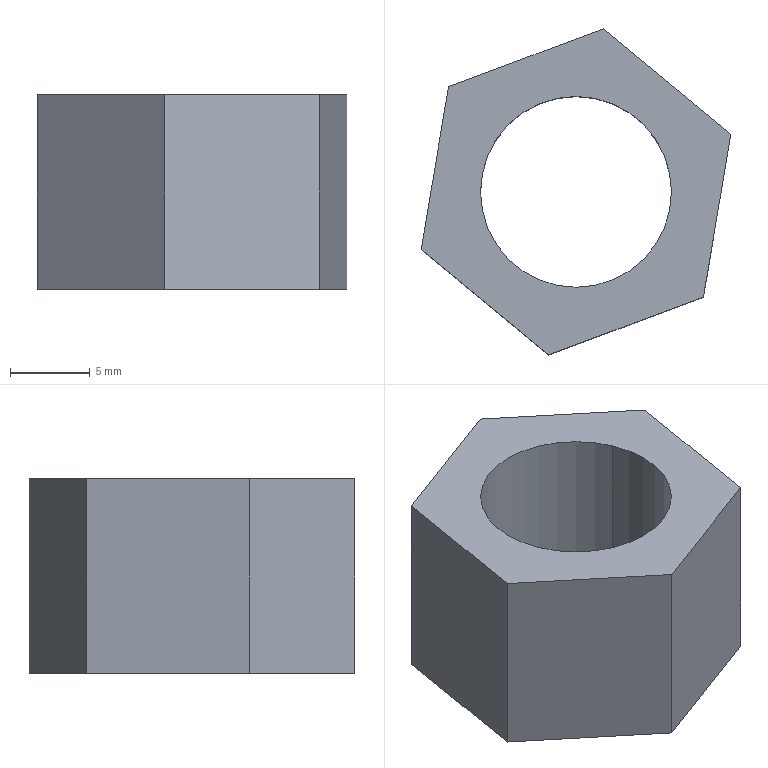Component | SolidWorks | M12Nut-2 | 1 solid | 10 faces | box 19.47 x 20.5 x 12.2 mm | volume 2043 mm3 | plane 8 | cylinder 2 | commonest cylinder face diameters 12 x2
STEP:
#1=COLOUR_RGB('',0.7922,0.8196,0.9333);
#2=FILL_AREA_STYLE_COLOUR('',#1);
#3=FILL_AREA_STYLE('',(#2));
#4=SURFACE_STYLE_FILL_AREA(#3);
#5=SURFACE_SIDE_STYLE('',(#4));
#6=SURFACE_STYLE_USAGE(.BOTH.,#5);
#7=PRESENTATION_STYLE_ASSIGNMENT((#6));
#8=CARTESIAN_POINT('',(21.066,-0.0173,0.542));
#9=VERTEX_POINT('',#8);
#10=CARTESIAN_POINT('',(20.629,-0.1983,0.542));
#11=VERTEX_POINT('',#10);
#12=CARTESIAN_POINT('',(20.847,-0.1078,0.542));
#13=DIRECTION('',(-0.,-0.,-1.));
#14=DIRECTION('',(-0.9237,-0.383,0.));
#15=AXIS2_PLACEMENT_3D('',#12,#13,#14);
#16=CIRCLE('',#15,0.2362);
#17=EDGE_CURVE('',#9,#11,#16,.T.);
#18=ORIENTED_EDGE('',*,*,#17,.F.);
#19=CARTESIAN_POINT('',(21.066,-0.0173,0.06171));
#20=VERTEX_POINT('',#19);
#21=CARTESIAN_POINT('',(21.066,-0.0173,0.5639));
#22=DIRECTION('',(-0.,-0.,-1.));
#23=VECTOR('',#22,39.37);
#24=LINE('',#21,#23);
#25=EDGE_CURVE('',#9,#20,#24,.T.);
#26=ORIENTED_EDGE('',*,*,#25,.T.);
#27=CARTESIAN_POINT('',(20.629,-0.1983,0.06171));
#28=VERTEX_POINT('',#27);
#29=CARTESIAN_POINT('',(20.847,-0.1078,0.06171));
#30=DIRECTION('',(-0.,-0.,-1.));
#31=DIRECTION('',(-0.9237,-0.383,0.));
#32=AXIS2_PLACEMENT_3D('',#29,#30,#31);
#33=CIRCLE('',#32,0.2362);
#34=EDGE_CURVE('',#20,#28,#33,.T.);
#35=ORIENTED_EDGE('',*,*,#34,.T.);
#36=CARTESIAN_POINT('',(20.629,-0.1983,0.5639));
#37=DIRECTION('',(-0.,-0.,-1.));
#38=VECTOR('',#37,39.37);
#39=LINE('',#36,#38);
#40=EDGE_CURVE('',#11,#28,#39,.T.);
#41=ORIENTED_EDGE('',*,*,#40,.F.);
#42=EDGE_LOOP('',(#18,#26,#35,#41));
#43=FACE_OUTER_BOUND('',#42,.T.);
#44=CARTESIAN_POINT('',(20.847,-0.1078,0.5639));
#45=DIRECTION('',(-0.,-0.,-1.));
#46=DIRECTION('',(-0.9237,-0.383,0.));
#47=AXIS2_PLACEMENT_3D('',#44,#45,#46);
#48=CYLINDRICAL_SURFACE('',#47,0.2362);
#49=ADVANCED_FACE('',(#43),#48,.F.);
#50=CARTESIAN_POINT('',(21.163,-0.3682,0.542));
#51=VERTEX_POINT('',#50);
#52=CARTESIAN_POINT('',(20.78,-0.5113,0.542));
#53=VERTEX_POINT('',#52);
#54=CARTESIAN_POINT('',(21.163,-0.3682,0.542));
#55=DIRECTION('',(-0.9369,-0.3497,0.));
#56=VECTOR('',#55,39.37);
#57=LINE('',#54,#56);
#58=EDGE_CURVE('',#51,#53,#57,.T.);
#59=ORIENTED_EDGE('',*,*,#58,.T.);
#60=CARTESIAN_POINT('',(20.78,-0.5113,0.06171));
#61=VERTEX_POINT('',#60);
#62=CARTESIAN_POINT('',(20.78,-0.5113,0.06171));
#63=DIRECTION('',(0.,0.,1.));
#64=VECTOR('',#63,39.37);
#65=LINE('',#62,#64);
#66=EDGE_CURVE('',#61,#53,#65,.T.);
#67=ORIENTED_EDGE('',*,*,#66,.F.);
#68=CARTESIAN_POINT('',(21.163,-0.3682,0.06171));
#69=VERTEX_POINT('',#68);
#70=CARTESIAN_POINT('',(21.163,-0.3682,0.06171));
#71=DIRECTION('',(-0.9369,-0.3497,0.));
#72=VECTOR('',#71,39.37);
#73=LINE('',#70,#72);
#74=EDGE_CURVE('',#69,#61,#73,.T.);
#75=ORIENTED_EDGE('',*,*,#74,.F.);
#76=CARTESIAN_POINT('',(21.163,-0.3682,0.06171));
#77=DIRECTION('',(0.,0.,1.));
#78=VECTOR('',#77,39.37);
#79=LINE('',#76,#78);
#80=EDGE_CURVE('',#69,#51,#79,.T.);
#81=ORIENTED_EDGE('',*,*,#80,.T.);
#82=EDGE_LOOP('',(#59,#67,#75,#81));
#83=FACE_OUTER_BOUND('',#82,.T.);
#84=CARTESIAN_POINT('',(21.163,-0.3682,0.06171));
#85=DIRECTION('',(-0.3497,0.9369,0.));
#86=DIRECTION('',(0.9369,0.3497,-0.));
#87=AXIS2_PLACEMENT_3D('',#84,#85,#86);
#88=PLANE('',#87);
#89=ADVANCED_FACE('',(#83),#88,.F.);
#90=CARTESIAN_POINT('',(20.464,-0.2509,0.542));
#91=VERTEX_POINT('',#90);
#92=CARTESIAN_POINT('',(20.78,-0.5113,0.542));
#93=DIRECTION('',(-0.7713,0.6365,0.));
#94=VECTOR('',#93,39.37);
#95=LINE('',#92,#94);
#96=EDGE_CURVE('',#53,#91,#95,.T.);
#97=ORIENTED_EDGE('',*,*,#96,.T.);
#98=CARTESIAN_POINT('',(20.464,-0.2509,0.06171));
#99=VERTEX_POINT('',#98);
#100=CARTESIAN_POINT('',(20.464,-0.2509,0.06171));
#101=DIRECTION('',(0.,0.,1.));
#102=VECTOR('',#101,39.37);
#103=LINE('',#100,#102);
#104=EDGE_CURVE('',#99,#91,#103,.T.);
#105=ORIENTED_EDGE('',*,*,#104,.F.);
#106=CARTESIAN_POINT('',(20.78,-0.5113,0.06171));
#107=DIRECTION('',(-0.7713,0.6365,0.));
#108=VECTOR('',#107,39.37);
#109=LINE('',#106,#108);
#110=EDGE_CURVE('',#61,#99,#109,.T.);
#111=ORIENTED_EDGE('',*,*,#110,.F.);
#112=ORIENTED_EDGE('',*,*,#66,.T.);
#113=EDGE_LOOP('',(#97,#105,#111,#112));
#114=FACE_OUTER_BOUND('',#113,.T.);
#115=CARTESIAN_POINT('',(20.78,-0.5113,0.06171));
#116=DIRECTION('',(0.6365,0.7713,-0.));
#117=DIRECTION('',(0.7713,-0.6365,-0.));
#118=AXIS2_PLACEMENT_3D('',#115,#116,#117);
#119=PLANE('',#118);
#120=ADVANCED_FACE('',(#114),#119,.F.);
#121=CARTESIAN_POINT('',(20.532,0.1526,0.542));
#122=VERTEX_POINT('',#121);
#123=CARTESIAN_POINT('',(20.464,-0.2509,0.542));
#124=DIRECTION('',(0.1656,0.9862,-0.));
#125=VECTOR('',#124,39.37);
#126=LINE('',#123,#125);
#127=EDGE_CURVE('',#91,#122,#126,.T.);
#128=ORIENTED_EDGE('',*,*,#127,.T.);
#129=CARTESIAN_POINT('',(20.532,0.1526,0.06171));
#130=VERTEX_POINT('',#129);
#131=CARTESIAN_POINT('',(20.532,0.1526,0.06171));
#132=DIRECTION('',(0.,0.,1.));
#133=VECTOR('',#132,39.37);
#134=LINE('',#131,#133);
#135=EDGE_CURVE('',#130,#122,#134,.T.);
#136=ORIENTED_EDGE('',*,*,#135,.F.);
#137=CARTESIAN_POINT('',(20.464,-0.2509,0.06171));
#138=DIRECTION('',(0.1656,0.9862,-0.));
#139=VECTOR('',#138,39.37);
#140=LINE('',#137,#139);
#141=EDGE_CURVE('',#99,#130,#140,.T.);
#142=ORIENTED_EDGE('',*,*,#141,.F.);
#143=ORIENTED_EDGE('',*,*,#104,.T.);
#144=EDGE_LOOP('',(#128,#136,#142,#143));
#145=FACE_OUTER_BOUND('',#144,.T.);
#146=CARTESIAN_POINT('',(20.464,-0.2509,0.06171));
#147=DIRECTION('',(0.9862,-0.1656,-0.));
#148=DIRECTION('',(-0.1656,-0.9862,0.));
#149=AXIS2_PLACEMENT_3D('',#146,#147,#148);
#150=PLANE('',#149);
#151=ADVANCED_FACE('',(#145),#150,.F.);
#152=CARTESIAN_POINT('',(20.915,0.2957,0.542));
#153=VERTEX_POINT('',#152);
#154=CARTESIAN_POINT('',(20.532,0.1526,0.542));
#155=DIRECTION('',(0.9369,0.3497,-0.));
#156=VECTOR('',#155,39.37);
#157=LINE('',#154,#156);
#158=EDGE_CURVE('',#122,#153,#157,.T.);
#159=ORIENTED_EDGE('',*,*,#158,.T.);
#160=CARTESIAN_POINT('',(20.915,0.2957,0.06171));
#161=VERTEX_POINT('',#160);
#162=CARTESIAN_POINT('',(20.915,0.2957,0.06171));
#163=DIRECTION('',(0.,0.,1.));
#164=VECTOR('',#163,39.37);
#165=LINE('',#162,#164);
#166=EDGE_CURVE('',#161,#153,#165,.T.);
#167=ORIENTED_EDGE('',*,*,#166,.F.);
#168=CARTESIAN_POINT('',(20.532,0.1526,0.06171));
#169=DIRECTION('',(0.9369,0.3497,-0.));
#170=VECTOR('',#169,39.37);
#171=LINE('',#168,#170);
#172=EDGE_CURVE('',#130,#161,#171,.T.);
#173=ORIENTED_EDGE('',*,*,#172,.F.);
#174=ORIENTED_EDGE('',*,*,#135,.T.);
#175=EDGE_LOOP('',(#159,#167,#173,#174));
#176=FACE_OUTER_BOUND('',#175,.T.);
#177=CARTESIAN_POINT('',(20.532,0.1526,0.06171));
#178=DIRECTION('',(0.3497,-0.9369,-0.));
#179=DIRECTION('',(-0.9369,-0.3497,0.));
#180=AXIS2_PLACEMENT_3D('',#177,#178,#179);
#181=PLANE('',#180);
#182=ADVANCED_FACE('',(#176),#181,.F.);
#183=CARTESIAN_POINT('',(21.231,0.03529,0.542));
#184=VERTEX_POINT('',#183);
#185=CARTESIAN_POINT('',(20.915,0.2957,0.542));
#186=DIRECTION('',(0.7713,-0.6365,-0.));
#187=VECTOR('',#186,39.37);
#188=LINE('',#185,#187);
#189=EDGE_CURVE('',#153,#184,#188,.T.);
#190=ORIENTED_EDGE('',*,*,#189,.T.);
#191=CARTESIAN_POINT('',(21.231,0.03529,0.06171));
#192=VERTEX_POINT('',#191);
#193=CARTESIAN_POINT('',(21.231,0.03529,0.06171));
#194=DIRECTION('',(0.,0.,1.));
#195=VECTOR('',#194,39.37);
#196=LINE('',#193,#195);
#197=EDGE_CURVE('',#192,#184,#196,.T.);
#198=ORIENTED_EDGE('',*,*,#197,.F.);
#199=CARTESIAN_POINT('',(20.915,0.2957,0.06171));
#200=DIRECTION('',(0.7713,-0.6365,-0.));
#201=VECTOR('',#200,39.37);
#202=LINE('',#199,#201);
#203=EDGE_CURVE('',#161,#192,#202,.T.);
#204=ORIENTED_EDGE('',*,*,#203,.F.);
#205=ORIENTED_EDGE('',*,*,#166,.T.);
#206=EDGE_LOOP('',(#190,#198,#204,#205));
#207=FACE_OUTER_BOUND('',#206,.T.);
#208=CARTESIAN_POINT('',(20.915,0.2957,0.06171));
#209=DIRECTION('',(-0.6365,-0.7713,0.));
#210=DIRECTION('',(-0.7713,0.6365,0.));
#211=AXIS2_PLACEMENT_3D('',#208,#209,#210);
#212=PLANE('',#211);
#213=ADVANCED_FACE('',(#207),#212,.F.);
#214=CARTESIAN_POINT('',(21.231,0.03529,0.542));
#215=DIRECTION('',(-0.1656,-0.9862,0.));
#216=VECTOR('',#215,39.37);
#217=LINE('',#214,#216);
#218=EDGE_CURVE('',#184,#51,#217,.T.);
#219=ORIENTED_EDGE('',*,*,#218,.T.);
#220=ORIENTED_EDGE('',*,*,#80,.F.);
#221=CARTESIAN_POINT('',(21.231,0.03529,0.06171));
#222=DIRECTION('',(-0.1656,-0.9862,0.));
#223=VECTOR('',#222,39.37);
#224=LINE('',#221,#223);
#225=EDGE_CURVE('',#192,#69,#224,.T.);
#226=ORIENTED_EDGE('',*,*,#225,.F.);
#227=ORIENTED_EDGE('',*,*,#197,.T.);
#228=EDGE_LOOP('',(#219,#220,#226,#227));
#229=FACE_OUTER_BOUND('',#228,.T.);
#230=CARTESIAN_POINT('',(21.231,0.03529,0.06171));
#231=DIRECTION('',(-0.9862,0.1656,0.));
#232=DIRECTION('',(0.1656,0.9862,-0.));
#233=AXIS2_PLACEMENT_3D('',#230,#231,#232);
#234=PLANE('',#233);
#235=ADVANCED_FACE('',(#229),#234,.F.);
#236=CARTESIAN_POINT('',(20.847,-0.1078,0.06171));
#237=DIRECTION('',(-0.,-0.,-1.));
#238=DIRECTION('',(-0.9237,-0.383,0.));
#239=AXIS2_PLACEMENT_3D('',#236,#237,#238);
#240=CIRCLE('',#239,0.2362);
#241=EDGE_CURVE('',#28,#20,#240,.T.);
#242=ORIENTED_EDGE('',*,*,#241,.F.);
#243=ORIENTED_EDGE('',*,*,#34,.F.);
#244=EDGE_LOOP('',(#242,#243));
#245=FACE_BOUND('',#244,.T.);
#246=ORIENTED_EDGE('',*,*,#74,.T.);
#247=ORIENTED_EDGE('',*,*,#110,.T.);
#248=ORIENTED_EDGE('',*,*,#141,.T.);
#249=ORIENTED_EDGE('',*,*,#172,.T.);
#250=ORIENTED_EDGE('',*,*,#203,.T.);
#251=ORIENTED_EDGE('',*,*,#225,.T.);
#252=EDGE_LOOP('',(#246,#247,#248,#249,#250,#251));
#253=FACE_OUTER_BOUND('',#252,.T.);
#254=CARTESIAN_POINT('',(21.086,-0.6843,0.06171));
#255=DIRECTION('',(-0.,-0.,-1.));
#256=DIRECTION('',(-0.9237,-0.383,0.));
#257=AXIS2_PLACEMENT_3D('',#254,#255,#256);
#258=PLANE('',#257);
#259=ADVANCED_FACE('',(#245,#253),#258,.T.);
#260=CARTESIAN_POINT('',(20.847,-0.1078,0.542));
#261=DIRECTION('',(-0.,-0.,-1.));
#262=DIRECTION('',(-0.9237,-0.383,0.));
#263=AXIS2_PLACEMENT_3D('',#260,#261,#262);
#264=CIRCLE('',#263,0.2362);
#265=EDGE_CURVE('',#11,#9,#264,.T.);
#266=ORIENTED_EDGE('',*,*,#265,.T.);
#267=ORIENTED_EDGE('',*,*,#17,.T.);
#268=EDGE_LOOP('',(#266,#267));
#269=FACE_BOUND('',#268,.T.);
#270=ORIENTED_EDGE('',*,*,#58,.F.);
#271=ORIENTED_EDGE('',*,*,#218,.F.);
#272=ORIENTED_EDGE('',*,*,#189,.F.);
#273=ORIENTED_EDGE('',*,*,#158,.F.);
#274=ORIENTED_EDGE('',*,*,#127,.F.);
#275=ORIENTED_EDGE('',*,*,#96,.F.);
#276=EDGE_LOOP('',(#270,#271,#272,#273,#274,#275));
#277=FACE_OUTER_BOUND('',#276,.T.);
#278=CARTESIAN_POINT('',(21.086,-0.6843,0.542));
#279=DIRECTION('',(-0.,-0.,-1.));
#280=DIRECTION('',(-0.9237,-0.383,0.));
#281=AXIS2_PLACEMENT_3D('',#278,#279,#280);
#282=PLANE('',#281);
#283=ADVANCED_FACE('',(#269,#277),#282,.F.);
#284=ORIENTED_EDGE('',*,*,#25,.F.);
#285=ORIENTED_EDGE('',*,*,#265,.F.);
#286=ORIENTED_EDGE('',*,*,#40,.T.);
#287=ORIENTED_EDGE('',*,*,#241,.T.);
#288=EDGE_LOOP('',(#284,#285,#286,#287));
#289=FACE_OUTER_BOUND('',#288,.T.);
#290=CARTESIAN_POINT('',(20.847,-0.1078,0.5639));
#291=DIRECTION('',(-0.,-0.,-1.));
#292=DIRECTION('',(-0.9237,-0.383,0.));
#293=AXIS2_PLACEMENT_3D('',#290,#291,#292);
#294=CYLINDRICAL_SURFACE('',#293,0.2362);
#295=ADVANCED_FACE('',(#289),#294,.F.);
#296=CLOSED_SHELL('',(#49,#89,#120,#151,#182,#213,#235,#259,#283,#295));
#297=MANIFOLD_SOLID_BREP('',#296);
#298=STYLED_ITEM('',(#7),#297);
#299=PRESENTATION_LAYER_ASSIGNMENT('','',(#298));
#300=(LENGTH_UNIT()NAMED_UNIT(*)SI_UNIT($,.METRE.));
#301=LENGTH_MEASURE_WITH_UNIT(LENGTH_MEASURE(0.0254),#300);
#302=DIMENSIONAL_EXPONENTS(1.,0.,0.,0.,0.,0.,0.);
#303=(CONVERSION_BASED_UNIT('',#301)LENGTH_UNIT()NAMED_UNIT(#302));
#304=UNCERTAINTY_MEASURE_WITH_UNIT(LENGTH_MEASURE(0.00001),#303,'','');
#305=(NAMED_UNIT(*)PLANE_ANGLE_UNIT()SI_UNIT($,.RADIAN.));
#306=(NAMED_UNIT(*)SI_UNIT($,.STERADIAN.)SOLID_ANGLE_UNIT());
#307=(GEOMETRIC_REPRESENTATION_CONTEXT(3)GLOBAL_UNCERTAINTY_ASSIGNED_CONTEXT((#304))GLOBAL_UNIT_ASSIGNED_CONTEXT((#303,#305,#306))REPRESENTATION_CONTEXT('',''));
#308=MECHANICAL_DESIGN_GEOMETRIC_PRESENTATION_REPRESENTATION('',(#298),#307);
#309=CARTESIAN_POINT('',(0.,0.,0.));
#310=DIRECTION('',(0.,0.,1.));
#311=DIRECTION('',(1.,0.,0.));
#312=AXIS2_PLACEMENT_3D('',#309,#310,#311);
#313=(LENGTH_UNIT()NAMED_UNIT(*)SI_UNIT($,.METRE.));
#314=LENGTH_MEASURE_WITH_UNIT(LENGTH_MEASURE(0.0254),#313);
#315=DIMENSIONAL_EXPONENTS(1.,0.,0.,0.,0.,0.,0.);
#316=(CONVERSION_BASED_UNIT('',#314)LENGTH_UNIT()NAMED_UNIT(#315));
#317=UNCERTAINTY_MEASURE_WITH_UNIT(LENGTH_MEASURE(0.00001),#316,'','');
#318=(NAMED_UNIT(*)PLANE_ANGLE_UNIT()SI_UNIT($,.RADIAN.));
#319=(NAMED_UNIT(*)SI_UNIT($,.STERADIAN.)SOLID_ANGLE_UNIT());
#320=(GEOMETRIC_REPRESENTATION_CONTEXT(3)GLOBAL_UNCERTAINTY_ASSIGNED_CONTEXT((#317))GLOBAL_UNIT_ASSIGNED_CONTEXT((#316,#318,#319))REPRESENTATION_CONTEXT('',''));
#321=ADVANCED_BREP_SHAPE_REPRESENTATION('',(#297,#312),#320);